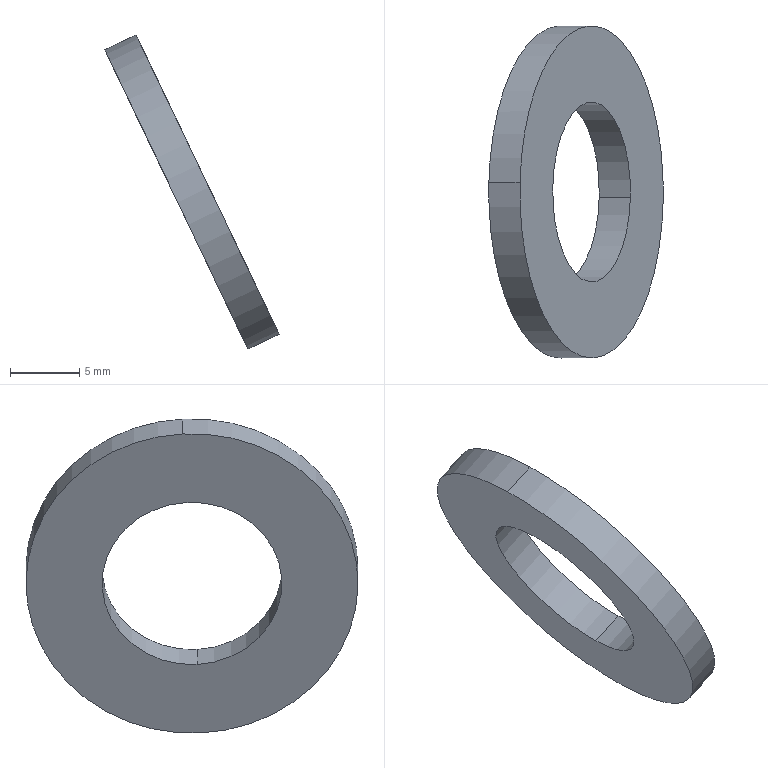Component | SolidWorks | plain washers-n series-grade a gb-1 | 1 solid | 6 faces | box 12.62 x 24 x 22.73 mm | volume 799 mm3 | cylinder 4 | plane 2 | commonest cylinder face diameters 13 x2 24 x2
build123d program:
from build123d import *

# Parameters (mm, degrees)
SKETCH1_R          = 12
SKETCH1_R_2        = 6.5
BASE_EXTRUDE_DEPTH = 2.5


with BuildPart() as part:
    # Sketch1 → Base-Extrude (new body)
    with BuildSketch(Plane.XY):
        Circle(SKETCH1_R)
        Circle(SKETCH1_R_2, mode=Mode.SUBTRACT)
    extrude(amount=-BASE_EXTRUDE_DEPTH)


solid = part.part

# Placed as in the assembly
solid = solid.moved(Location((37.842, 250, 476.494), (0, 64.419, 13.953)))
STEP:
#1=COLOUR_RGB('',0.7922,0.8196,0.9333);
#2=FILL_AREA_STYLE_COLOUR('',#1);
#3=FILL_AREA_STYLE('',(#2));
#4=SURFACE_STYLE_FILL_AREA(#3);
#5=SURFACE_SIDE_STYLE('',(#4));
#6=SURFACE_STYLE_USAGE(.BOTH.,#5);
#7=PRESENTATION_STYLE_ASSIGNMENT((#6));
#8=CARTESIAN_POINT('',(1.6,9.828,18.529));
#9=VERTEX_POINT('',#8);
#10=CARTESIAN_POINT('',(1.38,9.857,18.99));
#11=VERTEX_POINT('',#10);
#12=CARTESIAN_POINT('',(1.49,9.843,18.76));
#13=DIRECTION('',(-0.902,0.,-0.4318));
#14=DIRECTION('',(-0.4311,0.05587,0.9006));
#15=AXIS2_PLACEMENT_3D('',#12,#13,#14);
#16=CIRCLE('',#15,0.2559);
#17=EDGE_CURVE('',#9,#11,#16,.T.);
#18=ORIENTED_EDGE('',*,*,#17,.F.);
#19=CARTESIAN_POINT('',(1.511,9.828,18.487));
#20=VERTEX_POINT('',#19);
#21=CARTESIAN_POINT('',(1.6,9.828,18.529));
#22=DIRECTION('',(-0.902,0.,-0.4318));
#23=VECTOR('',#22,39.37);
#24=LINE('',#21,#23);
#25=EDGE_CURVE('',#9,#20,#24,.T.);
#26=ORIENTED_EDGE('',*,*,#25,.T.);
#27=CARTESIAN_POINT('',(1.291,9.857,18.948));
#28=VERTEX_POINT('',#27);
#29=CARTESIAN_POINT('',(1.401,9.843,18.717));
#30=DIRECTION('',(-0.902,0.,-0.4318));
#31=DIRECTION('',(-0.4311,0.05587,0.9006));
#32=AXIS2_PLACEMENT_3D('',#29,#30,#31);
#33=CIRCLE('',#32,0.2559);
#34=EDGE_CURVE('',#20,#28,#33,.T.);
#35=ORIENTED_EDGE('',*,*,#34,.T.);
#36=CARTESIAN_POINT('',(1.38,9.857,18.99));
#37=DIRECTION('',(-0.902,0.,-0.4318));
#38=VECTOR('',#37,39.37);
#39=LINE('',#36,#38);
#40=EDGE_CURVE('',#11,#28,#39,.T.);
#41=ORIENTED_EDGE('',*,*,#40,.F.);
#42=EDGE_LOOP('',(#18,#26,#35,#41));
#43=FACE_OUTER_BOUND('',#42,.T.);
#44=CARTESIAN_POINT('',(1.49,9.843,18.76));
#45=DIRECTION('',(-0.902,0.,-0.4318));
#46=DIRECTION('',(-0.4311,0.05587,0.9006));
#47=AXIS2_PLACEMENT_3D('',#44,#45,#46);
#48=CYLINDRICAL_SURFACE('',#47,0.2559);
#49=ADVANCED_FACE('',(#43),#48,.F.);
#50=CARTESIAN_POINT('',(1.286,9.869,19.185));
#51=VERTEX_POINT('',#50);
#52=CARTESIAN_POINT('',(1.694,9.816,18.334));
#53=VERTEX_POINT('',#52);
#54=CARTESIAN_POINT('',(1.49,9.843,18.76));
#55=DIRECTION('',(-0.902,0.,-0.4318));
#56=DIRECTION('',(-0.4311,0.05587,0.9006));
#57=AXIS2_PLACEMENT_3D('',#54,#55,#56);
#58=CIRCLE('',#57,0.4724);
#59=EDGE_CURVE('',#51,#53,#58,.T.);
#60=ORIENTED_EDGE('',*,*,#59,.T.);
#61=CARTESIAN_POINT('',(1.605,9.816,18.292));
#62=VERTEX_POINT('',#61);
#63=CARTESIAN_POINT('',(1.694,9.816,18.334));
#64=DIRECTION('',(-0.902,0.,-0.4318));
#65=VECTOR('',#64,39.37);
#66=LINE('',#63,#65);
#67=EDGE_CURVE('',#53,#62,#66,.T.);
#68=ORIENTED_EDGE('',*,*,#67,.T.);
#69=CARTESIAN_POINT('',(1.197,9.869,19.143));
#70=VERTEX_POINT('',#69);
#71=CARTESIAN_POINT('',(1.401,9.843,18.717));
#72=DIRECTION('',(-0.902,0.,-0.4318));
#73=DIRECTION('',(-0.4311,0.05587,0.9006));
#74=AXIS2_PLACEMENT_3D('',#71,#72,#73);
#75=CIRCLE('',#74,0.4724);
#76=EDGE_CURVE('',#70,#62,#75,.T.);
#77=ORIENTED_EDGE('',*,*,#76,.F.);
#78=CARTESIAN_POINT('',(1.286,9.869,19.185));
#79=DIRECTION('',(-0.902,0.,-0.4318));
#80=VECTOR('',#79,39.37);
#81=LINE('',#78,#80);
#82=EDGE_CURVE('',#51,#70,#81,.T.);
#83=ORIENTED_EDGE('',*,*,#82,.F.);
#84=EDGE_LOOP('',(#60,#68,#77,#83));
#85=FACE_OUTER_BOUND('',#84,.T.);
#86=CARTESIAN_POINT('',(1.49,9.843,18.76));
#87=DIRECTION('',(-0.902,0.,-0.4318));
#88=DIRECTION('',(-0.4311,0.05587,0.9006));
#89=AXIS2_PLACEMENT_3D('',#86,#87,#88);
#90=CYLINDRICAL_SURFACE('',#89,0.4724);
#91=ADVANCED_FACE('',(#85),#90,.T.);
#92=ORIENTED_EDGE('',*,*,#67,.F.);
#93=CARTESIAN_POINT('',(1.49,9.843,18.76));
#94=DIRECTION('',(-0.902,0.,-0.4318));
#95=DIRECTION('',(-0.4311,0.05587,0.9006));
#96=AXIS2_PLACEMENT_3D('',#93,#94,#95);
#97=CIRCLE('',#96,0.4724);
#98=EDGE_CURVE('',#53,#51,#97,.T.);
#99=ORIENTED_EDGE('',*,*,#98,.T.);
#100=ORIENTED_EDGE('',*,*,#82,.T.);
#101=CARTESIAN_POINT('',(1.401,9.843,18.717));
#102=DIRECTION('',(-0.902,0.,-0.4318));
#103=DIRECTION('',(-0.4311,0.05587,0.9006));
#104=AXIS2_PLACEMENT_3D('',#101,#102,#103);
#105=CIRCLE('',#104,0.4724);
#106=EDGE_CURVE('',#62,#70,#105,.T.);
#107=ORIENTED_EDGE('',*,*,#106,.F.);
#108=EDGE_LOOP('',(#92,#99,#100,#107));
#109=FACE_OUTER_BOUND('',#108,.T.);
#110=CARTESIAN_POINT('',(1.49,9.843,18.76));
#111=DIRECTION('',(-0.902,0.,-0.4318));
#112=DIRECTION('',(-0.4311,0.05587,0.9006));
#113=AXIS2_PLACEMENT_3D('',#110,#111,#112);
#114=CYLINDRICAL_SURFACE('',#113,0.4724);
#115=ADVANCED_FACE('',(#109),#114,.T.);
#116=CARTESIAN_POINT('',(1.49,9.843,18.76));
#117=DIRECTION('',(-0.902,0.,-0.4318));
#118=DIRECTION('',(-0.4311,0.05587,0.9006));
#119=AXIS2_PLACEMENT_3D('',#116,#117,#118);
#120=CIRCLE('',#119,0.2559);
#121=EDGE_CURVE('',#11,#9,#120,.T.);
#122=ORIENTED_EDGE('',*,*,#121,.T.);
#123=ORIENTED_EDGE('',*,*,#17,.T.);
#124=EDGE_LOOP('',(#122,#123));
#125=FACE_BOUND('',#124,.T.);
#126=ORIENTED_EDGE('',*,*,#59,.F.);
#127=ORIENTED_EDGE('',*,*,#98,.F.);
#128=EDGE_LOOP('',(#126,#127));
#129=FACE_OUTER_BOUND('',#128,.T.);
#130=CARTESIAN_POINT('',(1.49,9.843,18.76));
#131=DIRECTION('',(-0.902,0.,-0.4318));
#132=DIRECTION('',(-0.4311,0.05587,0.9006));
#133=AXIS2_PLACEMENT_3D('',#130,#131,#132);
#134=PLANE('',#133);
#135=ADVANCED_FACE('',(#125,#129),#134,.F.);
#136=CARTESIAN_POINT('',(1.401,9.843,18.717));
#137=DIRECTION('',(-0.902,0.,-0.4318));
#138=DIRECTION('',(-0.4311,0.05587,0.9006));
#139=AXIS2_PLACEMENT_3D('',#136,#137,#138);
#140=CIRCLE('',#139,0.2559);
#141=EDGE_CURVE('',#28,#20,#140,.T.);
#142=ORIENTED_EDGE('',*,*,#141,.F.);
#143=ORIENTED_EDGE('',*,*,#34,.F.);
#144=EDGE_LOOP('',(#142,#143));
#145=FACE_BOUND('',#144,.T.);
#146=ORIENTED_EDGE('',*,*,#76,.T.);
#147=ORIENTED_EDGE('',*,*,#106,.T.);
#148=EDGE_LOOP('',(#146,#147));
#149=FACE_OUTER_BOUND('',#148,.T.);
#150=CARTESIAN_POINT('',(1.401,9.843,18.717));
#151=DIRECTION('',(-0.902,0.,-0.4318));
#152=DIRECTION('',(-0.4311,0.05587,0.9006));
#153=AXIS2_PLACEMENT_3D('',#150,#151,#152);
#154=PLANE('',#153);
#155=ADVANCED_FACE('',(#145,#149),#154,.T.);
#156=ORIENTED_EDGE('',*,*,#25,.F.);
#157=ORIENTED_EDGE('',*,*,#121,.F.);
#158=ORIENTED_EDGE('',*,*,#40,.T.);
#159=ORIENTED_EDGE('',*,*,#141,.T.);
#160=EDGE_LOOP('',(#156,#157,#158,#159));
#161=FACE_OUTER_BOUND('',#160,.T.);
#162=CARTESIAN_POINT('',(1.49,9.843,18.76));
#163=DIRECTION('',(-0.902,0.,-0.4318));
#164=DIRECTION('',(-0.4311,0.05587,0.9006));
#165=AXIS2_PLACEMENT_3D('',#162,#163,#164);
#166=CYLINDRICAL_SURFACE('',#165,0.2559);
#167=ADVANCED_FACE('',(#161),#166,.F.);
#168=CLOSED_SHELL('',(#49,#91,#115,#135,#155,#167));
#169=MANIFOLD_SOLID_BREP('',#168);
#170=STYLED_ITEM('',(#7),#169);
#171=(LENGTH_UNIT()NAMED_UNIT(*)SI_UNIT($,.METRE.));
#172=LENGTH_MEASURE_WITH_UNIT(LENGTH_MEASURE(0.0254),#171);
#173=DIMENSIONAL_EXPONENTS(1.,0.,0.,0.,0.,0.,0.);
#174=(CONVERSION_BASED_UNIT('',#172)LENGTH_UNIT()NAMED_UNIT(#173));
#175=UNCERTAINTY_MEASURE_WITH_UNIT(LENGTH_MEASURE(0.00001),#174,'','');
#176=(NAMED_UNIT(*)PLANE_ANGLE_UNIT()SI_UNIT($,.RADIAN.));
#177=(NAMED_UNIT(*)SI_UNIT($,.STERADIAN.)SOLID_ANGLE_UNIT());
#178=(GEOMETRIC_REPRESENTATION_CONTEXT(3)GLOBAL_UNCERTAINTY_ASSIGNED_CONTEXT((#175))GLOBAL_UNIT_ASSIGNED_CONTEXT((#174,#176,#177))REPRESENTATION_CONTEXT('',''));
#179=MECHANICAL_DESIGN_GEOMETRIC_PRESENTATION_REPRESENTATION('',(#170),#178);
#180=PRESENTATION_LAYER_ASSIGNMENT('','',(#170));
#181=CARTESIAN_POINT('',(0.,0.,0.));
#182=DIRECTION('',(0.,0.,1.));
#183=DIRECTION('',(1.,0.,0.));
#184=AXIS2_PLACEMENT_3D('',#181,#182,#183);
#185=(LENGTH_UNIT()NAMED_UNIT(*)SI_UNIT($,.METRE.));
#186=LENGTH_MEASURE_WITH_UNIT(LENGTH_MEASURE(0.0254),#185);
#187=DIMENSIONAL_EXPONENTS(1.,0.,0.,0.,0.,0.,0.);
#188=(CONVERSION_BASED_UNIT('',#186)LENGTH_UNIT()NAMED_UNIT(#187));
#189=UNCERTAINTY_MEASURE_WITH_UNIT(LENGTH_MEASURE(0.00001),#188,'','');
#190=(NAMED_UNIT(*)PLANE_ANGLE_UNIT()SI_UNIT($,.RADIAN.));
#191=(NAMED_UNIT(*)SI_UNIT($,.STERADIAN.)SOLID_ANGLE_UNIT());
#192=(GEOMETRIC_REPRESENTATION_CONTEXT(3)GLOBAL_UNCERTAINTY_ASSIGNED_CONTEXT((#189))GLOBAL_UNIT_ASSIGNED_CONTEXT((#188,#190,#191))REPRESENTATION_CONTEXT('',''));
#193=ADVANCED_BREP_SHAPE_REPRESENTATION('',(#169,#184),#192);